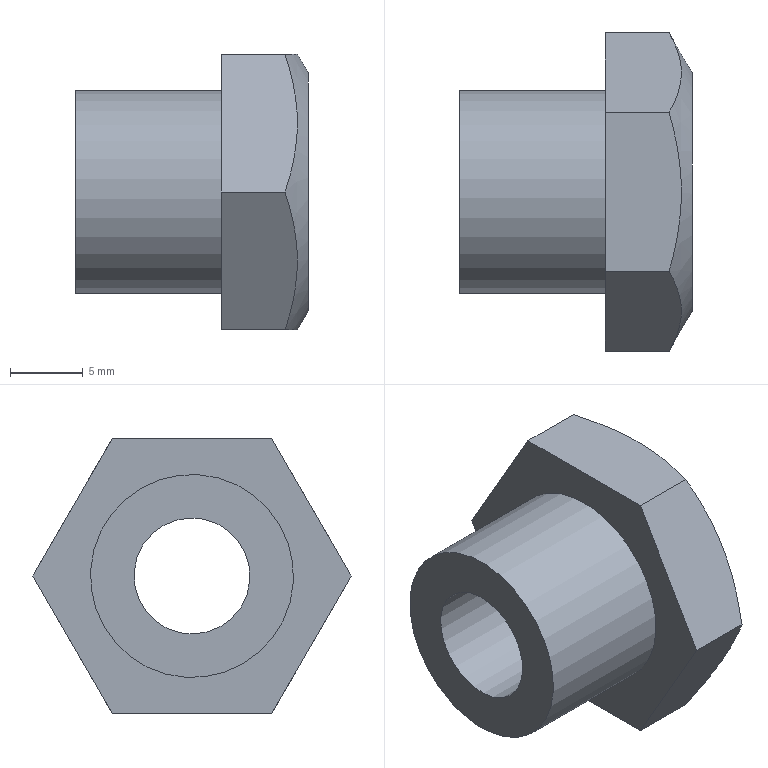Component | NX | OUTER_CASING_TUBE_CONNECTING_SCREW | 1 solid | 12 faces | box 16 x 21.94 x 19 mm | volume 2555 mm3 | plane 9 | cylinder 2 | cone 1 | commonest cylinder face diameters 14 x1 8 x1
STEP:
#1=CARTESIAN_POINT('',(0.,0.,0.));
#2=DIRECTION('',(0.,0.,1.));
#3=DIRECTION('',(1.,0.,0.));
#4=AXIS2_PLACEMENT_3D('',#1,#2,#3);
#5=CARTESIAN_POINT('',(-38.73,-48.,41.964));
#6=VERTEX_POINT('',#5);
#7=CARTESIAN_POINT('',(-38.73,-52.,35.036));
#8=VERTEX_POINT('',#7);
#9=CARTESIAN_POINT('',(-38.73,-50.,38.5));
#10=DIRECTION('',(1.,0.,0.));
#11=DIRECTION('',(0.,0.5,0.866));
#12=AXIS2_PLACEMENT_3D('',#9,#10,#11);
#13=CIRCLE('',#12,4.);
#14=CARTESIAN_POINT('',(-38.73,-50.,38.5));
#15=DIRECTION('',(-1.,0.,0.));
#16=DIRECTION('',(0.,0.5,0.866));
#17=AXIS2_PLACEMENT_3D('',#14,#15,#16);
#18=PLANE('',#17);
#19=CARTESIAN_POINT('',(4.,0.));
#20=CARTESIAN_POINT('',(4.,-6.928));
#21=CARTESIAN_POINT('',(-2.,-3.464));
#22=CARTESIAN_POINT('',(-8.,-0.));
#23=CARTESIAN_POINT('',(-2.,3.464));
#24=CARTESIAN_POINT('',(4.,6.928));
#25=CARTESIAN_POINT('',(4.,0.));
#26=(BOUNDED_CURVE()B_SPLINE_CURVE(2,(#19,#20,#21,#22,#23,#24,#25),.UNSPECIFIED.,.T.,.F.)B_SPLINE_CURVE_WITH_KNOTS((1,2,2,2,2,1),(-2.094,0.,2.094,4.189,6.283,8.378),.UNSPECIFIED.)CURVE()GEOMETRIC_REPRESENTATION_ITEM()RATIONAL_B_SPLINE_CURVE((1.,0.5,1.,0.5,1.,0.5,1.))REPRESENTATION_ITEM(''));
#27=(GEOMETRIC_REPRESENTATION_CONTEXT(2)PARAMETRIC_REPRESENTATION_CONTEXT()REPRESENTATION_CONTEXT('',''));
#28=DEFINITIONAL_REPRESENTATION('',(#26),#27);
#29=PCURVE('',#18,#28);
#30=CARTESIAN_POINT('',(-44.23,-50.,38.5));
#31=DIRECTION('',(1.,0.,0.));
#32=DIRECTION('',(0.,-0.5,-0.866));
#33=AXIS2_PLACEMENT_3D('',#30,#31,#32);
#34=CYLINDRICAL_SURFACE('',#33,4.);
#35=CARTESIAN_POINT('',(3.142,5.5));
#36=DIRECTION('',(1.,0.));
#37=VECTOR('',#36,1.);
#38=LINE('',#35,#37);
#39=(GEOMETRIC_REPRESENTATION_CONTEXT(2)PARAMETRIC_REPRESENTATION_CONTEXT()REPRESENTATION_CONTEXT('',''));
#40=DEFINITIONAL_REPRESENTATION('',(#38),#39);
#41=PCURVE('',#34,#40);
#42=SURFACE_CURVE('',#13,(#29,#41),.PCURVE_S1.);
#43=EDGE_CURVE('',#6,#8,#42,.T.);
#44=ORIENTED_EDGE('',*,*,#43,.T.);
#45=CARTESIAN_POINT('',(-38.73,-50.,38.5));
#46=DIRECTION('',(1.,0.,0.));
#47=DIRECTION('',(0.,0.5,0.866));
#48=AXIS2_PLACEMENT_3D('',#45,#46,#47);
#49=CIRCLE('',#48,4.);
#50=CARTESIAN_POINT('',(4.,0.));
#51=CARTESIAN_POINT('',(4.,-6.928));
#52=CARTESIAN_POINT('',(-2.,-3.464));
#53=CARTESIAN_POINT('',(-8.,-0.));
#54=CARTESIAN_POINT('',(-2.,3.464));
#55=CARTESIAN_POINT('',(4.,6.928));
#56=CARTESIAN_POINT('',(4.,0.));
#57=(BOUNDED_CURVE()B_SPLINE_CURVE(2,(#50,#51,#52,#53,#54,#55,#56),.UNSPECIFIED.,.T.,.F.)B_SPLINE_CURVE_WITH_KNOTS((1,2,2,2,2,1),(-2.094,0.,2.094,4.189,6.283,8.378),.UNSPECIFIED.)CURVE()GEOMETRIC_REPRESENTATION_ITEM()RATIONAL_B_SPLINE_CURVE((1.,0.5,1.,0.5,1.,0.5,1.))REPRESENTATION_ITEM(''));
#58=(GEOMETRIC_REPRESENTATION_CONTEXT(2)PARAMETRIC_REPRESENTATION_CONTEXT()REPRESENTATION_CONTEXT('',''));
#59=DEFINITIONAL_REPRESENTATION('',(#57),#58);
#60=PCURVE('',#18,#59);
#61=CARTESIAN_POINT('',(-3.142,5.5));
#62=DIRECTION('',(1.,0.));
#63=VECTOR('',#62,1.);
#64=LINE('',#61,#63);
#65=(GEOMETRIC_REPRESENTATION_CONTEXT(2)PARAMETRIC_REPRESENTATION_CONTEXT()REPRESENTATION_CONTEXT('',''));
#66=DEFINITIONAL_REPRESENTATION('',(#64),#65);
#67=PCURVE('',#34,#66);
#68=SURFACE_CURVE('',#49,(#60,#67),.PCURVE_S1.);
#69=EDGE_CURVE('',#8,#6,#68,.T.);
#70=ORIENTED_EDGE('',*,*,#69,.T.);
#71=EDGE_LOOP('',(#44,#70));
#72=FACE_BOUND('',#71,.T.);
#73=CARTESIAN_POINT('',(-38.73,-53.5,32.438));
#74=VERTEX_POINT('',#73);
#75=CARTESIAN_POINT('',(-38.73,-50.,38.5));
#76=DIRECTION('',(1.,0.,0.));
#77=DIRECTION('',(0.,-0.5,-0.866));
#78=AXIS2_PLACEMENT_3D('',#75,#76,#77);
#79=CIRCLE('',#78,7.);
#80=CARTESIAN_POINT('',(-7.,0.));
#81=CARTESIAN_POINT('',(-7.,12.124));
#82=CARTESIAN_POINT('',(3.5,6.062));
#83=CARTESIAN_POINT('',(14.,-0.));
#84=CARTESIAN_POINT('',(3.5,-6.062));
#85=CARTESIAN_POINT('',(-7.,-12.124));
#86=CARTESIAN_POINT('',(-7.,0.));
#87=(BOUNDED_CURVE()B_SPLINE_CURVE(2,(#80,#81,#82,#83,#84,#85,#86),.UNSPECIFIED.,.T.,.F.)B_SPLINE_CURVE_WITH_KNOTS((1,2,2,2,2,1),(-2.094,0.,2.094,4.189,6.283,8.378),.UNSPECIFIED.)CURVE()GEOMETRIC_REPRESENTATION_ITEM()RATIONAL_B_SPLINE_CURVE((1.,0.5,1.,0.5,1.,0.5,1.))REPRESENTATION_ITEM(''));
#88=(GEOMETRIC_REPRESENTATION_CONTEXT(2)PARAMETRIC_REPRESENTATION_CONTEXT()REPRESENTATION_CONTEXT('',''));
#89=DEFINITIONAL_REPRESENTATION('',(#87),#88);
#90=PCURVE('',#18,#89);
#91=CARTESIAN_POINT('',(-38.73,-50.,38.5));
#92=DIRECTION('',(1.,0.,0.));
#93=DIRECTION('',(0.,-0.5,-0.866));
#94=AXIS2_PLACEMENT_3D('',#91,#92,#93);
#95=CYLINDRICAL_SURFACE('',#94,7.);
#96=CARTESIAN_POINT('',(0.,0.));
#97=DIRECTION('',(1.,0.));
#98=VECTOR('',#97,1.);
#99=LINE('',#96,#98);
#100=(GEOMETRIC_REPRESENTATION_CONTEXT(2)PARAMETRIC_REPRESENTATION_CONTEXT()REPRESENTATION_CONTEXT('',''));
#101=DEFINITIONAL_REPRESENTATION('',(#99),#100);
#102=PCURVE('',#95,#101);
#103=SURFACE_CURVE('',#79,(#90,#102),.PCURVE_S1.);
#104=EDGE_CURVE('',#74,#74,#103,.T.);
#105=ORIENTED_EDGE('',*,*,#104,.F.);
#106=EDGE_LOOP('',(#105));
#107=FACE_BOUND('',#106,.T.);
#108=ADVANCED_FACE('',(#72,#107),#18,.T.);
#109=CARTESIAN_POINT('',(-28.73,-53.5,32.438));
#110=VERTEX_POINT('',#109);
#111=CARTESIAN_POINT('',(-28.73,-50.,38.5));
#112=DIRECTION('',(-1.,0.,0.));
#113=DIRECTION('',(0.,-0.5,-0.866));
#114=AXIS2_PLACEMENT_3D('',#111,#112,#113);
#115=CIRCLE('',#114,7.);
#116=CARTESIAN_POINT('',(6.283,10.));
#117=DIRECTION('',(-1.,0.));
#118=VECTOR('',#117,1.);
#119=LINE('',#116,#118);
#120=(GEOMETRIC_REPRESENTATION_CONTEXT(2)PARAMETRIC_REPRESENTATION_CONTEXT()REPRESENTATION_CONTEXT('',''));
#121=DEFINITIONAL_REPRESENTATION('',(#119),#120);
#122=PCURVE('',#95,#121);
#123=CARTESIAN_POINT('',(-28.73,-50.,38.5));
#124=DIRECTION('',(-1.,0.,0.));
#125=DIRECTION('',(0.,0.5,0.866));
#126=AXIS2_PLACEMENT_3D('',#123,#124,#125);
#127=PLANE('',#126);
#128=CARTESIAN_POINT('',(0.,0.));
#129=DIRECTION('',(-1.,0.));
#130=AXIS2_PLACEMENT_2D('',#128,#129);
#131=CIRCLE('',#130,7.);
#132=(GEOMETRIC_REPRESENTATION_CONTEXT(2)PARAMETRIC_REPRESENTATION_CONTEXT()REPRESENTATION_CONTEXT('',''));
#133=DEFINITIONAL_REPRESENTATION('',(#131),#132);
#134=PCURVE('',#127,#133);
#135=SURFACE_CURVE('',#115,(#122,#134),.PCURVE_S1.);
#136=EDGE_CURVE('',#110,#110,#135,.T.);
#137=ORIENTED_EDGE('',*,*,#136,.T.);
#138=CARTESIAN_POINT('',(-38.73,-53.5,32.438));
#139=CARTESIAN_POINT('',(-28.73,-53.5,32.438));
#140=B_SPLINE_CURVE_WITH_KNOTS('',1,(#138,#139),.UNSPECIFIED.,.F.,.F.,(2,2),(0.,10.),.PIECEWISE_BEZIER_KNOTS.);
#141=CARTESIAN_POINT('',(0.,0.));
#142=DIRECTION('',(0.,1.));
#143=VECTOR('',#142,1.);
#144=LINE('',#141,#143);
#145=(GEOMETRIC_REPRESENTATION_CONTEXT(2)PARAMETRIC_REPRESENTATION_CONTEXT()REPRESENTATION_CONTEXT('',''));
#146=DEFINITIONAL_REPRESENTATION('',(#144),#145);
#147=PCURVE('',#95,#146);
#148=CARTESIAN_POINT('',(6.283,0.));
#149=DIRECTION('',(0.,1.));
#150=VECTOR('',#149,1.);
#151=LINE('',#148,#150);
#152=(GEOMETRIC_REPRESENTATION_CONTEXT(2)PARAMETRIC_REPRESENTATION_CONTEXT()REPRESENTATION_CONTEXT('',''));
#153=DEFINITIONAL_REPRESENTATION('',(#151),#152);
#154=PCURVE('',#95,#153);
#155=SEAM_CURVE('',#140,(#147,#154),.PCURVE_S1.);
#156=EDGE_CURVE('',#74,#110,#155,.T.);
#157=ORIENTED_EDGE('',*,*,#156,.F.);
#158=ORIENTED_EDGE('',*,*,#104,.T.);
#159=ORIENTED_EDGE('',*,*,#156,.T.);
#160=EDGE_LOOP('',(#137,#157,#158,#159));
#161=FACE_BOUND('',#160,.T.);
#162=ADVANCED_FACE('',(#161),#95,.T.);
#163=CARTESIAN_POINT('',(-24.314,-55.485,29.));
#164=VERTEX_POINT('',#163);
#165=CARTESIAN_POINT('',(-24.314,-44.515,29.));
#166=VERTEX_POINT('',#165);
#167=CARTESIAN_POINT('',(-24.314,-55.485,29.));
#168=CARTESIAN_POINT('',(-23.797,-53.694,29.));
#169=CARTESIAN_POINT('',(-23.466,-51.876,29.));
#170=CARTESIAN_POINT('',(-23.464,-48.145,29.));
#171=CARTESIAN_POINT('',(-23.796,-46.309,29.));
#172=CARTESIAN_POINT('',(-24.314,-44.515,29.));
#173=B_SPLINE_CURVE_WITH_KNOTS('',3,(#167,#168,#169,#170,#171,#172),.UNSPECIFIED.,.F.,.F.,(4,2,4),(0.,0.5,1.),.UNSPECIFIED.);
#174=CARTESIAN_POINT('',(-22.73,-44.515,29.));
#175=DIRECTION('',(0.,0.,-1.));
#176=DIRECTION('',(0.,1.,0.));
#177=AXIS2_PLACEMENT_3D('',#174,#175,#176);
#178=PLANE('',#177);
#179=CARTESIAN_POINT('',(-10.97,-1.583));
#180=CARTESIAN_POINT('',(-9.179,-1.066));
#181=CARTESIAN_POINT('',(-7.361,-0.736));
#182=CARTESIAN_POINT('',(-3.63,-0.7336));
#183=CARTESIAN_POINT('',(-1.793,-1.066));
#184=CARTESIAN_POINT('',(0.,-1.583));
#185=B_SPLINE_CURVE_WITH_KNOTS('',3,(#179,#180,#181,#182,#183,#184),.UNSPECIFIED.,.F.,.F.,(4,2,4),(0.,0.5,1.),.UNSPECIFIED.);
#186=(GEOMETRIC_REPRESENTATION_CONTEXT(2)PARAMETRIC_REPRESENTATION_CONTEXT()REPRESENTATION_CONTEXT('',''));
#187=DEFINITIONAL_REPRESENTATION('',(#185),#186);
#188=PCURVE('',#178,#187);
#189=CARTESIAN_POINT('',(-22.73,-50.,38.5));
#190=DIRECTION('',(-1.,0.,0.));
#191=DIRECTION('',(0.,0.5,0.866));
#192=AXIS2_PLACEMENT_3D('',#189,#190,#191);
#193=CONICAL_SURFACE('',#192,8.227,1.047);
#194=CARTESIAN_POINT('',(3.142,1.583));
#195=CARTESIAN_POINT('',(3.129,1.536));
#196=CARTESIAN_POINT('',(3.102,1.445));
#197=CARTESIAN_POINT('',(3.061,1.319));
#198=CARTESIAN_POINT('',(3.018,1.202));
#199=CARTESIAN_POINT('',(2.973,1.097));
#200=CARTESIAN_POINT('',(2.926,1.004));
#201=CARTESIAN_POINT('',(2.878,0.9237));
#202=CARTESIAN_POINT('',(2.828,0.8564));
#203=CARTESIAN_POINT('',(2.777,0.8031));
#204=CARTESIAN_POINT('',(2.725,0.7642));
#205=CARTESIAN_POINT('',(2.673,0.7404));
#206=CARTESIAN_POINT('',(2.619,0.7322));
#207=CARTESIAN_POINT('',(2.566,0.7398));
#208=CARTESIAN_POINT('',(2.513,0.7631));
#209=CARTESIAN_POINT('',(2.46,0.8015));
#210=CARTESIAN_POINT('',(2.409,0.8547));
#211=CARTESIAN_POINT('',(2.359,0.9219));
#212=CARTESIAN_POINT('',(2.311,1.003));
#213=CARTESIAN_POINT('',(2.264,1.096));
#214=CARTESIAN_POINT('',(2.218,1.201));
#215=CARTESIAN_POINT('',(2.175,1.318));
#216=CARTESIAN_POINT('',(2.134,1.445));
#217=CARTESIAN_POINT('',(2.107,1.536));
#218=CARTESIAN_POINT('',(2.094,1.583));
#219=B_SPLINE_CURVE_WITH_KNOTS('',3,(#194,#195,#196,#197,#198,#199,#200,#201,#202,#203,#204,#205,#206,#207,#208,#209,#210,#211,#212,#213,#214,#215,#216,#217,#218),.UNSPECIFIED.,.F.,.F.,(4,1,1,1,1,1,1,1,1,1,1,1,1,1,1,1,1,1,1,1,1,1,4),(0.,0.04545,0.09091,0.1364,0.1818,0.2273,0.2727,0.3182,0.3636,0.4091,0.4545,0.5,0.5455,0.5909,0.6364,0.6818,0.7273,0.7727,0.8182,0.8636,0.9091,0.9545,1.),.QUASI_UNIFORM_KNOTS.);
#220=(GEOMETRIC_REPRESENTATION_CONTEXT(2)PARAMETRIC_REPRESENTATION_CONTEXT()REPRESENTATION_CONTEXT('',''));
#221=DEFINITIONAL_REPRESENTATION('',(#219),#220);
#222=PCURVE('',#193,#221);
#223=SURFACE_CURVE('',#173,(#188,#222),.PCURVE_S1.);
#224=EDGE_CURVE('',#164,#166,#223,.T.);
#225=ORIENTED_EDGE('',*,*,#224,.F.);
#226=CARTESIAN_POINT('',(-28.73,-55.485,29.));
#227=VERTEX_POINT('',#226);
#228=CARTESIAN_POINT('',(-22.73,-55.485,29.));
#229=DIRECTION('',(-1.,0.,0.));
#230=VECTOR('',#229,1.);
#231=LINE('',#228,#230);
#232=CARTESIAN_POINT('',(-10.97,0.));
#233=DIRECTION('',(0.,-1.));
#234=VECTOR('',#233,1.);
#235=LINE('',#232,#234);
#236=(GEOMETRIC_REPRESENTATION_CONTEXT(2)PARAMETRIC_REPRESENTATION_CONTEXT()REPRESENTATION_CONTEXT('',''));
#237=DEFINITIONAL_REPRESENTATION('',(#235),#236);
#238=PCURVE('',#178,#237);
#239=CARTESIAN_POINT('',(-22.73,-55.485,29.));
#240=DIRECTION('',(0.,-0.866,-0.5));
#241=DIRECTION('',(0.,0.5,-0.866));
#242=AXIS2_PLACEMENT_3D('',#239,#240,#241);
#243=PLANE('',#242);
#244=CARTESIAN_POINT('',(0.,0.));
#245=DIRECTION('',(0.,-1.));
#246=VECTOR('',#245,1.);
#247=LINE('',#244,#246);
#248=(GEOMETRIC_REPRESENTATION_CONTEXT(2)PARAMETRIC_REPRESENTATION_CONTEXT()REPRESENTATION_CONTEXT('',''));
#249=DEFINITIONAL_REPRESENTATION('',(#247),#248);
#250=PCURVE('',#243,#249);
#251=SURFACE_CURVE('',#231,(#238,#250),.PCURVE_S1.);
#252=EDGE_CURVE('',#164,#227,#251,.T.);
#253=ORIENTED_EDGE('',*,*,#252,.T.);
#254=CARTESIAN_POINT('',(-28.73,-44.515,29.));
#255=VERTEX_POINT('',#254);
#256=CARTESIAN_POINT('',(-28.73,-44.515,29.));
#257=DIRECTION('',(0.,-1.,-0.));
#258=VECTOR('',#257,1.);
#259=LINE('',#256,#258);
#260=CARTESIAN_POINT('',(0.,-6.));
#261=DIRECTION('',(-1.,0.));
#262=VECTOR('',#261,1.);
#263=LINE('',#260,#262);
#264=(GEOMETRIC_REPRESENTATION_CONTEXT(2)PARAMETRIC_REPRESENTATION_CONTEXT()REPRESENTATION_CONTEXT('',''));
#265=DEFINITIONAL_REPRESENTATION('',(#263),#264);
#266=PCURVE('',#178,#265);
#267=CARTESIAN_POINT('',(-5.485,9.5));
#268=DIRECTION('',(-0.5,-0.866));
#269=VECTOR('',#268,1.);
#270=LINE('',#267,#269);
#271=(GEOMETRIC_REPRESENTATION_CONTEXT(2)PARAMETRIC_REPRESENTATION_CONTEXT()REPRESENTATION_CONTEXT('',''));
#272=DEFINITIONAL_REPRESENTATION('',(#270),#271);
#273=PCURVE('',#127,#272);
#274=SURFACE_CURVE('',#259,(#266,#273),.PCURVE_S1.);
#275=EDGE_CURVE('',#255,#227,#274,.T.);
#276=ORIENTED_EDGE('',*,*,#275,.F.);
#277=CARTESIAN_POINT('',(-22.73,-44.515,29.));
#278=DIRECTION('',(-1.,0.,0.));
#279=VECTOR('',#278,1.);
#280=LINE('',#277,#279);
#281=CARTESIAN_POINT('',(0.,0.));
#282=DIRECTION('',(0.,-1.));
#283=VECTOR('',#282,1.);
#284=LINE('',#281,#283);
#285=(GEOMETRIC_REPRESENTATION_CONTEXT(2)PARAMETRIC_REPRESENTATION_CONTEXT()REPRESENTATION_CONTEXT('',''));
#286=DEFINITIONAL_REPRESENTATION('',(#284),#285);
#287=PCURVE('',#178,#286);
#288=CARTESIAN_POINT('',(-22.73,-39.03,38.5));
#289=DIRECTION('',(0.,0.866,-0.5));
#290=DIRECTION('',(0.,0.5,0.866));
#291=AXIS2_PLACEMENT_3D('',#288,#289,#290);
#292=PLANE('',#291);
#293=CARTESIAN_POINT('',(-10.97,0.));
#294=DIRECTION('',(0.,-1.));
#295=VECTOR('',#294,1.);
#296=LINE('',#293,#295);
#297=(GEOMETRIC_REPRESENTATION_CONTEXT(2)PARAMETRIC_REPRESENTATION_CONTEXT()REPRESENTATION_CONTEXT('',''));
#298=DEFINITIONAL_REPRESENTATION('',(#296),#297);
#299=PCURVE('',#292,#298);
#300=SURFACE_CURVE('',#280,(#287,#299),.PCURVE_S1.);
#301=EDGE_CURVE('',#166,#255,#300,.T.);
#302=ORIENTED_EDGE('',*,*,#301,.F.);
#303=EDGE_LOOP('',(#225,#253,#276,#302));
#304=FACE_BOUND('',#303,.T.);
#305=ADVANCED_FACE('',(#304),#178,.T.);
#306=CARTESIAN_POINT('',(-24.314,-60.97,38.5));
#307=VERTEX_POINT('',#306);
#308=CARTESIAN_POINT('',(-24.314,-60.97,38.5));
#309=CARTESIAN_POINT('',(-23.797,-60.074,36.949));
#310=CARTESIAN_POINT('',(-23.466,-59.165,35.374));
#311=CARTESIAN_POINT('',(-23.464,-57.3,32.144));
#312=CARTESIAN_POINT('',(-23.796,-56.382,30.553));
#313=CARTESIAN_POINT('',(-24.314,-55.485,29.));
#314=B_SPLINE_CURVE_WITH_KNOTS('',3,(#308,#309,#310,#311,#312,#313),.UNSPECIFIED.,.F.,.F.,(4,2,4),(0.,0.5,1.),.UNSPECIFIED.);
#315=CARTESIAN_POINT('',(-10.97,-1.583));
#316=CARTESIAN_POINT('',(-9.179,-1.066));
#317=CARTESIAN_POINT('',(-7.361,-0.736));
#318=CARTESIAN_POINT('',(-3.63,-0.7336));
#319=CARTESIAN_POINT('',(-1.793,-1.066));
#320=CARTESIAN_POINT('',(0.,-1.583));
#321=B_SPLINE_CURVE_WITH_KNOTS('',3,(#315,#316,#317,#318,#319,#320),.UNSPECIFIED.,.F.,.F.,(4,2,4),(0.,0.5,1.),.UNSPECIFIED.);
#322=(GEOMETRIC_REPRESENTATION_CONTEXT(2)PARAMETRIC_REPRESENTATION_CONTEXT()REPRESENTATION_CONTEXT('',''));
#323=DEFINITIONAL_REPRESENTATION('',(#321),#322);
#324=PCURVE('',#243,#323);
#325=CARTESIAN_POINT('',(4.189,1.583));
#326=CARTESIAN_POINT('',(4.176,1.536));
#327=CARTESIAN_POINT('',(4.15,1.445));
#328=CARTESIAN_POINT('',(4.108,1.319));
#329=CARTESIAN_POINT('',(4.065,1.202));
#330=CARTESIAN_POINT('',(4.02,1.097));
#331=CARTESIAN_POINT('',(3.974,1.004));
#332=CARTESIAN_POINT('',(3.925,0.9237));
#333=CARTESIAN_POINT('',(3.876,0.8564));
#334=CARTESIAN_POINT('',(3.825,0.8031));
#335=CARTESIAN_POINT('',(3.773,0.7642));
#336=CARTESIAN_POINT('',(3.72,0.7404));
#337=CARTESIAN_POINT('',(3.666,0.7322));
#338=CARTESIAN_POINT('',(3.613,0.7398));
#339=CARTESIAN_POINT('',(3.56,0.7631));
#340=CARTESIAN_POINT('',(3.507,0.8015));
#341=CARTESIAN_POINT('',(3.456,0.8547));
#342=CARTESIAN_POINT('',(3.406,0.9219));
#343=CARTESIAN_POINT('',(3.358,1.003));
#344=CARTESIAN_POINT('',(3.311,1.096));
#345=CARTESIAN_POINT('',(3.266,1.201));
#346=CARTESIAN_POINT('',(3.222,1.318));
#347=CARTESIAN_POINT('',(3.181,1.445));
#348=CARTESIAN_POINT('',(3.154,1.536));
#349=CARTESIAN_POINT('',(3.142,1.583));
#350=B_SPLINE_CURVE_WITH_KNOTS('',3,(#325,#326,#327,#328,#329,#330,#331,#332,#333,#334,#335,#336,#337,#338,#339,#340,#341,#342,#343,#344,#345,#346,#347,#348,#349),.UNSPECIFIED.,.F.,.F.,(4,1,1,1,1,1,1,1,1,1,1,1,1,1,1,1,1,1,1,1,1,1,4),(0.,0.04545,0.09091,0.1364,0.1818,0.2273,0.2727,0.3182,0.3636,0.4091,0.4545,0.5,0.5455,0.5909,0.6364,0.6818,0.7273,0.7727,0.8182,0.8636,0.9091,0.9545,1.),.QUASI_UNIFORM_KNOTS.);
#351=(GEOMETRIC_REPRESENTATION_CONTEXT(2)PARAMETRIC_REPRESENTATION_CONTEXT()REPRESENTATION_CONTEXT('',''));
#352=DEFINITIONAL_REPRESENTATION('',(#350),#351);
#353=PCURVE('',#193,#352);
#354=SURFACE_CURVE('',#314,(#324,#353),.PCURVE_S1.);
#355=EDGE_CURVE('',#307,#164,#354,.T.);
#356=ORIENTED_EDGE('',*,*,#355,.F.);
#357=CARTESIAN_POINT('',(-28.73,-60.97,38.5));
#358=VERTEX_POINT('',#357);
#359=CARTESIAN_POINT('',(-22.73,-60.97,38.5));
#360=DIRECTION('',(-1.,0.,0.));
#361=VECTOR('',#360,1.);
#362=LINE('',#359,#361);
#363=CARTESIAN_POINT('',(-10.97,0.));
#364=DIRECTION('',(0.,-1.));
#365=VECTOR('',#364,1.);
#366=LINE('',#363,#365);
#367=(GEOMETRIC_REPRESENTATION_CONTEXT(2)PARAMETRIC_REPRESENTATION_CONTEXT()REPRESENTATION_CONTEXT('',''));
#368=DEFINITIONAL_REPRESENTATION('',(#366),#367);
#369=PCURVE('',#243,#368);
#370=CARTESIAN_POINT('',(-22.73,-60.97,38.5));
#371=DIRECTION('',(0.,-0.866,0.5));
#372=DIRECTION('',(0.,-0.5,-0.866));
#373=AXIS2_PLACEMENT_3D('',#370,#371,#372);
#374=PLANE('',#373);
#375=CARTESIAN_POINT('',(0.,0.));
#376=DIRECTION('',(0.,-1.));
#377=VECTOR('',#376,1.);
#378=LINE('',#375,#377);
#379=(GEOMETRIC_REPRESENTATION_CONTEXT(2)PARAMETRIC_REPRESENTATION_CONTEXT()REPRESENTATION_CONTEXT('',''));
#380=DEFINITIONAL_REPRESENTATION('',(#378),#379);
#381=PCURVE('',#374,#380);
#382=SURFACE_CURVE('',#362,(#369,#381),.PCURVE_S1.);
#383=EDGE_CURVE('',#307,#358,#382,.T.);
#384=ORIENTED_EDGE('',*,*,#383,.T.);
#385=CARTESIAN_POINT('',(-28.73,-55.485,29.));
#386=DIRECTION('',(0.,-0.5,0.866));
#387=VECTOR('',#386,1.);
#388=LINE('',#385,#387);
#389=CARTESIAN_POINT('',(0.,-6.));
#390=DIRECTION('',(-1.,0.));
#391=VECTOR('',#390,1.);
#392=LINE('',#389,#391);
#393=(GEOMETRIC_REPRESENTATION_CONTEXT(2)PARAMETRIC_REPRESENTATION_CONTEXT()REPRESENTATION_CONTEXT('',''));
#394=DEFINITIONAL_REPRESENTATION('',(#392),#393);
#395=PCURVE('',#243,#394);
#396=CARTESIAN_POINT('',(-10.97,0.));
#397=DIRECTION('',(0.5,-0.866));
#398=VECTOR('',#397,1.);
#399=LINE('',#396,#398);
#400=(GEOMETRIC_REPRESENTATION_CONTEXT(2)PARAMETRIC_REPRESENTATION_CONTEXT()REPRESENTATION_CONTEXT('',''));
#401=DEFINITIONAL_REPRESENTATION('',(#399),#400);
#402=PCURVE('',#127,#401);
#403=SURFACE_CURVE('',#388,(#395,#402),.PCURVE_S1.);
#404=EDGE_CURVE('',#227,#358,#403,.T.);
#405=ORIENTED_EDGE('',*,*,#404,.F.);
#406=ORIENTED_EDGE('',*,*,#252,.F.);
#407=EDGE_LOOP('',(#356,#384,#405,#406));
#408=FACE_BOUND('',#407,.T.);
#409=ADVANCED_FACE('',(#408),#243,.T.);
#410=CARTESIAN_POINT('',(-24.314,-55.485,48.));
#411=VERTEX_POINT('',#410);
#412=CARTESIAN_POINT('',(-24.314,-55.485,48.));
#413=CARTESIAN_POINT('',(-23.799,-56.377,46.455));
#414=CARTESIAN_POINT('',(-23.465,-57.301,44.854));
#415=CARTESIAN_POINT('',(-23.465,-59.155,41.643));
#416=CARTESIAN_POINT('',(-23.802,-60.083,40.036));
#417=CARTESIAN_POINT('',(-24.314,-60.97,38.5));
#418=B_SPLINE_CURVE_WITH_KNOTS('',3,(#412,#413,#414,#415,#416,#417),.UNSPECIFIED.,.F.,.F.,(4,2,4),(0.,0.5,1.),.UNSPECIFIED.);
#419=CARTESIAN_POINT('',(-10.97,-1.583));
#420=CARTESIAN_POINT('',(-9.186,-1.068));
#421=CARTESIAN_POINT('',(-7.337,-0.7347));
#422=CARTESIAN_POINT('',(-3.63,-0.735));
#423=CARTESIAN_POINT('',(-1.773,-1.071));
#424=CARTESIAN_POINT('',(0.,-1.583));
#425=B_SPLINE_CURVE_WITH_KNOTS('',3,(#419,#420,#421,#422,#423,#424),.UNSPECIFIED.,.F.,.F.,(4,2,4),(0.,0.5,1.),.UNSPECIFIED.);
#426=(GEOMETRIC_REPRESENTATION_CONTEXT(2)PARAMETRIC_REPRESENTATION_CONTEXT()REPRESENTATION_CONTEXT('',''));
#427=DEFINITIONAL_REPRESENTATION('',(#425),#426);
#428=PCURVE('',#374,#427);
#429=CARTESIAN_POINT('',(5.236,1.583));
#430=CARTESIAN_POINT('',(5.223,1.537));
#431=CARTESIAN_POINT('',(5.197,1.446));
#432=CARTESIAN_POINT('',(5.156,1.319));
#433=CARTESIAN_POINT('',(5.112,1.202));
#434=CARTESIAN_POINT('',(5.067,1.097));
#435=CARTESIAN_POINT('',(5.02,1.003));
#436=CARTESIAN_POINT('',(4.972,0.9227));
#437=CARTESIAN_POINT('',(4.922,0.8553));
#438=CARTESIAN_POINT('',(4.87,0.802));
#439=CARTESIAN_POINT('',(4.818,0.7634));
#440=CARTESIAN_POINT('',(4.765,0.74));
#441=CARTESIAN_POINT('',(4.712,0.7322));
#442=CARTESIAN_POINT('',(4.659,0.7402));
#443=CARTESIAN_POINT('',(4.606,0.7637));
#444=CARTESIAN_POINT('',(4.554,0.8025));
#445=CARTESIAN_POINT('',(4.503,0.856));
#446=CARTESIAN_POINT('',(4.453,0.9236));
#447=CARTESIAN_POINT('',(4.404,1.005));
#448=CARTESIAN_POINT('',(4.357,1.098));
#449=CARTESIAN_POINT('',(4.312,1.204));
#450=CARTESIAN_POINT('',(4.269,1.32));
#451=CARTESIAN_POINT('',(4.228,1.446));
#452=CARTESIAN_POINT('',(4.202,1.537));
#453=CARTESIAN_POINT('',(4.189,1.583));
#454=B_SPLINE_CURVE_WITH_KNOTS('',3,(#429,#430,#431,#432,#433,#434,#435,#436,#437,#438,#439,#440,#441,#442,#443,#444,#445,#446,#447,#448,#449,#450,#451,#452,#453),.UNSPECIFIED.,.F.,.F.,(4,1,1,1,1,1,1,1,1,1,1,1,1,1,1,1,1,1,1,1,1,1,4),(0.,0.04545,0.09091,0.1364,0.1818,0.2273,0.2727,0.3182,0.3636,0.4091,0.4545,0.5,0.5455,0.5909,0.6364,0.6818,0.7273,0.7727,0.8182,0.8636,0.9091,0.9545,1.),.QUASI_UNIFORM_KNOTS.);
#455=(GEOMETRIC_REPRESENTATION_CONTEXT(2)PARAMETRIC_REPRESENTATION_CONTEXT()REPRESENTATION_CONTEXT('',''));
#456=DEFINITIONAL_REPRESENTATION('',(#454),#455);
#457=PCURVE('',#193,#456);
#458=SURFACE_CURVE('',#418,(#428,#457),.PCURVE_S1.);
#459=EDGE_CURVE('',#411,#307,#458,.T.);
#460=ORIENTED_EDGE('',*,*,#459,.F.);
#461=CARTESIAN_POINT('',(-28.73,-55.485,48.));
#462=VERTEX_POINT('',#461);
#463=CARTESIAN_POINT('',(-22.73,-55.485,48.));
#464=DIRECTION('',(-1.,0.,0.));
#465=VECTOR('',#464,1.);
#466=LINE('',#463,#465);
#467=CARTESIAN_POINT('',(-10.97,0.));
#468=DIRECTION('',(0.,-1.));
#469=VECTOR('',#468,1.);
#470=LINE('',#467,#469);
#471=(GEOMETRIC_REPRESENTATION_CONTEXT(2)PARAMETRIC_REPRESENTATION_CONTEXT()REPRESENTATION_CONTEXT('',''));
#472=DEFINITIONAL_REPRESENTATION('',(#470),#471);
#473=PCURVE('',#374,#472);
#474=CARTESIAN_POINT('',(-22.73,-55.485,48.));
#475=DIRECTION('',(0.,-0.,1.));
#476=DIRECTION('',(0.,-1.,-0.));
#477=AXIS2_PLACEMENT_3D('',#474,#475,#476);
#478=PLANE('',#477);
#479=CARTESIAN_POINT('',(0.,0.));
#480=DIRECTION('',(0.,-1.));
#481=VECTOR('',#480,1.);
#482=LINE('',#479,#481);
#483=(GEOMETRIC_REPRESENTATION_CONTEXT(2)PARAMETRIC_REPRESENTATION_CONTEXT()REPRESENTATION_CONTEXT('',''));
#484=DEFINITIONAL_REPRESENTATION('',(#482),#483);
#485=PCURVE('',#478,#484);
#486=SURFACE_CURVE('',#466,(#473,#485),.PCURVE_S1.);
#487=EDGE_CURVE('',#411,#462,#486,.T.);
#488=ORIENTED_EDGE('',*,*,#487,.T.);
#489=CARTESIAN_POINT('',(-28.73,-60.97,38.5));
#490=DIRECTION('',(0.,0.5,0.866));
#491=VECTOR('',#490,1.);
#492=LINE('',#489,#491);
#493=CARTESIAN_POINT('',(0.,-6.));
#494=DIRECTION('',(-1.,0.));
#495=VECTOR('',#494,1.);
#496=LINE('',#493,#495);
#497=(GEOMETRIC_REPRESENTATION_CONTEXT(2)PARAMETRIC_REPRESENTATION_CONTEXT()REPRESENTATION_CONTEXT('',''));
#498=DEFINITIONAL_REPRESENTATION('',(#496),#497);
#499=PCURVE('',#374,#498);
#500=CARTESIAN_POINT('',(-5.485,-9.5));
#501=DIRECTION('',(1.,0.));
#502=VECTOR('',#501,1.);
#503=LINE('',#500,#502);
#504=(GEOMETRIC_REPRESENTATION_CONTEXT(2)PARAMETRIC_REPRESENTATION_CONTEXT()REPRESENTATION_CONTEXT('',''));
#505=DEFINITIONAL_REPRESENTATION('',(#503),#504);
#506=PCURVE('',#127,#505);
#507=SURFACE_CURVE('',#492,(#499,#506),.PCURVE_S1.);
#508=EDGE_CURVE('',#358,#462,#507,.T.);
#509=ORIENTED_EDGE('',*,*,#508,.F.);
#510=ORIENTED_EDGE('',*,*,#383,.F.);
#511=EDGE_LOOP('',(#460,#488,#509,#510));
#512=FACE_BOUND('',#511,.T.);
#513=ADVANCED_FACE('',(#512),#374,.T.);
#514=CARTESIAN_POINT('',(-24.314,-44.515,48.));
#515=VERTEX_POINT('',#514);
#516=CARTESIAN_POINT('',(-24.314,-44.515,48.));
#517=CARTESIAN_POINT('',(-23.797,-46.306,48.));
#518=CARTESIAN_POINT('',(-23.466,-48.124,48.));
#519=CARTESIAN_POINT('',(-23.464,-51.855,48.));
#520=CARTESIAN_POINT('',(-23.796,-53.691,48.));
#521=CARTESIAN_POINT('',(-24.314,-55.485,48.));
#522=B_SPLINE_CURVE_WITH_KNOTS('',3,(#516,#517,#518,#519,#520,#521),.UNSPECIFIED.,.F.,.F.,(4,2,4),(0.,0.5,1.),.UNSPECIFIED.);
#523=CARTESIAN_POINT('',(-10.97,-1.583));
#524=CARTESIAN_POINT('',(-9.179,-1.066));
#525=CARTESIAN_POINT('',(-7.361,-0.736));
#526=CARTESIAN_POINT('',(-3.63,-0.7336));
#527=CARTESIAN_POINT('',(-1.793,-1.066));
#528=CARTESIAN_POINT('',(0.,-1.583));
#529=B_SPLINE_CURVE_WITH_KNOTS('',3,(#523,#524,#525,#526,#527,#528),.UNSPECIFIED.,.F.,.F.,(4,2,4),(0.,0.5,1.),.UNSPECIFIED.);
#530=(GEOMETRIC_REPRESENTATION_CONTEXT(2)PARAMETRIC_REPRESENTATION_CONTEXT()REPRESENTATION_CONTEXT('',''));
#531=DEFINITIONAL_REPRESENTATION('',(#529),#530);
#532=PCURVE('',#478,#531);
#533=CARTESIAN_POINT('',(6.283,1.583));
#534=CARTESIAN_POINT('',(6.27,1.536));
#535=CARTESIAN_POINT('',(6.244,1.445));
#536=CARTESIAN_POINT('',(6.203,1.319));
#537=CARTESIAN_POINT('',(6.16,1.202));
#538=CARTESIAN_POINT('',(6.115,1.097));
#539=CARTESIAN_POINT('',(6.068,1.004));
#540=CARTESIAN_POINT('',(6.02,0.9237));
#541=CARTESIAN_POINT('',(5.97,0.8564));
#542=CARTESIAN_POINT('',(5.919,0.8031));
#543=CARTESIAN_POINT('',(5.867,0.7642));
#544=CARTESIAN_POINT('',(5.814,0.7404));
#545=CARTESIAN_POINT('',(5.761,0.7322));
#546=CARTESIAN_POINT('',(5.707,0.7398));
#547=CARTESIAN_POINT('',(5.654,0.7631));
#548=CARTESIAN_POINT('',(5.602,0.8015));
#549=CARTESIAN_POINT('',(5.551,0.8547));
#550=CARTESIAN_POINT('',(5.501,0.9219));
#551=CARTESIAN_POINT('',(5.452,1.003));
#552=CARTESIAN_POINT('',(5.405,1.096));
#553=CARTESIAN_POINT('',(5.36,1.201));
#554=CARTESIAN_POINT('',(5.317,1.318));
#555=CARTESIAN_POINT('',(5.275,1.445));
#556=CARTESIAN_POINT('',(5.249,1.536));
#557=CARTESIAN_POINT('',(5.236,1.583));
#558=B_SPLINE_CURVE_WITH_KNOTS('',3,(#533,#534,#535,#536,#537,#538,#539,#540,#541,#542,#543,#544,#545,#546,#547,#548,#549,#550,#551,#552,#553,#554,#555,#556,#557),.UNSPECIFIED.,.F.,.F.,(4,1,1,1,1,1,1,1,1,1,1,1,1,1,1,1,1,1,1,1,1,1,4),(0.,0.04545,0.09091,0.1364,0.1818,0.2273,0.2727,0.3182,0.3636,0.4091,0.4545,0.5,0.5455,0.5909,0.6364,0.6818,0.7273,0.7727,0.8182,0.8636,0.9091,0.9545,1.),.QUASI_UNIFORM_KNOTS.);
#559=(GEOMETRIC_REPRESENTATION_CONTEXT(2)PARAMETRIC_REPRESENTATION_CONTEXT()REPRESENTATION_CONTEXT('',''));
#560=DEFINITIONAL_REPRESENTATION('',(#558),#559);
#561=PCURVE('',#193,#560);
#562=SURFACE_CURVE('',#522,(#532,#561),.PCURVE_S1.);
#563=EDGE_CURVE('',#515,#411,#562,.T.);
#564=ORIENTED_EDGE('',*,*,#563,.F.);
#565=CARTESIAN_POINT('',(-28.73,-44.515,48.));
#566=VERTEX_POINT('',#565);
#567=CARTESIAN_POINT('',(-22.73,-44.515,48.));
#568=DIRECTION('',(-1.,0.,0.));
#569=VECTOR('',#568,1.);
#570=LINE('',#567,#569);
#571=CARTESIAN_POINT('',(-10.97,0.));
#572=DIRECTION('',(0.,-1.));
#573=VECTOR('',#572,1.);
#574=LINE('',#571,#573);
#575=(GEOMETRIC_REPRESENTATION_CONTEXT(2)PARAMETRIC_REPRESENTATION_CONTEXT()REPRESENTATION_CONTEXT('',''));
#576=DEFINITIONAL_REPRESENTATION('',(#574),#575);
#577=PCURVE('',#478,#576);
#578=CARTESIAN_POINT('',(-22.73,-44.515,48.));
#579=DIRECTION('',(0.,0.866,0.5));
#580=DIRECTION('',(0.,-0.5,0.866));
#581=AXIS2_PLACEMENT_3D('',#578,#579,#580);
#582=PLANE('',#581);
#583=CARTESIAN_POINT('',(0.,0.));
#584=DIRECTION('',(0.,-1.));
#585=VECTOR('',#584,1.);
#586=LINE('',#583,#585);
#587=(GEOMETRIC_REPRESENTATION_CONTEXT(2)PARAMETRIC_REPRESENTATION_CONTEXT()REPRESENTATION_CONTEXT('',''));
#588=DEFINITIONAL_REPRESENTATION('',(#586),#587);
#589=PCURVE('',#582,#588);
#590=SURFACE_CURVE('',#570,(#577,#589),.PCURVE_S1.);
#591=EDGE_CURVE('',#515,#566,#590,.T.);
#592=ORIENTED_EDGE('',*,*,#591,.T.);
#593=CARTESIAN_POINT('',(-28.73,-55.485,48.));
#594=DIRECTION('',(0.,1.,0.));
#595=VECTOR('',#594,1.);
#596=LINE('',#593,#595);
#597=CARTESIAN_POINT('',(0.,-6.));
#598=DIRECTION('',(-1.,0.));
#599=VECTOR('',#598,1.);
#600=LINE('',#597,#599);
#601=(GEOMETRIC_REPRESENTATION_CONTEXT(2)PARAMETRIC_REPRESENTATION_CONTEXT()REPRESENTATION_CONTEXT('',''));
#602=DEFINITIONAL_REPRESENTATION('',(#600),#601);
#603=PCURVE('',#478,#602);
#604=CARTESIAN_POINT('',(5.485,-9.5));
#605=DIRECTION('',(0.5,0.866));
#606=VECTOR('',#605,1.);
#607=LINE('',#604,#606);
#608=(GEOMETRIC_REPRESENTATION_CONTEXT(2)PARAMETRIC_REPRESENTATION_CONTEXT()REPRESENTATION_CONTEXT('',''));
#609=DEFINITIONAL_REPRESENTATION('',(#607),#608);
#610=PCURVE('',#127,#609);
#611=SURFACE_CURVE('',#596,(#603,#610),.PCURVE_S1.);
#612=EDGE_CURVE('',#462,#566,#611,.T.);
#613=ORIENTED_EDGE('',*,*,#612,.F.);
#614=ORIENTED_EDGE('',*,*,#487,.F.);
#615=EDGE_LOOP('',(#564,#592,#613,#614));
#616=FACE_BOUND('',#615,.T.);
#617=ADVANCED_FACE('',(#616),#478,.T.);
#618=CARTESIAN_POINT('',(-24.314,-39.03,38.5));
#619=VERTEX_POINT('',#618);
#620=CARTESIAN_POINT('',(-24.314,-39.03,38.5));
#621=CARTESIAN_POINT('',(-23.797,-39.926,40.051));
#622=CARTESIAN_POINT('',(-23.466,-40.835,41.626));
#623=CARTESIAN_POINT('',(-23.464,-42.7,44.856));
#624=CARTESIAN_POINT('',(-23.796,-43.618,46.447));
#625=CARTESIAN_POINT('',(-24.314,-44.515,48.));
#626=B_SPLINE_CURVE_WITH_KNOTS('',3,(#620,#621,#622,#623,#624,#625),.UNSPECIFIED.,.F.,.F.,(4,2,4),(0.,0.5,1.),.UNSPECIFIED.);
#627=CARTESIAN_POINT('',(-10.97,-1.583));
#628=CARTESIAN_POINT('',(-9.179,-1.066));
#629=CARTESIAN_POINT('',(-7.361,-0.736));
#630=CARTESIAN_POINT('',(-3.63,-0.7336));
#631=CARTESIAN_POINT('',(-1.793,-1.066));
#632=CARTESIAN_POINT('',(0.,-1.583));
#633=B_SPLINE_CURVE_WITH_KNOTS('',3,(#627,#628,#629,#630,#631,#632),.UNSPECIFIED.,.F.,.F.,(4,2,4),(0.,0.5,1.),.UNSPECIFIED.);
#634=(GEOMETRIC_REPRESENTATION_CONTEXT(2)PARAMETRIC_REPRESENTATION_CONTEXT()REPRESENTATION_CONTEXT('',''));
#635=DEFINITIONAL_REPRESENTATION('',(#633),#634);
#636=PCURVE('',#582,#635);
#637=CARTESIAN_POINT('',(1.047,1.583));
#638=CARTESIAN_POINT('',(1.034,1.536));
#639=CARTESIAN_POINT('',(1.008,1.445));
#640=CARTESIAN_POINT('',(0.9667,1.319));
#641=CARTESIAN_POINT('',(0.9236,1.202));
#642=CARTESIAN_POINT('',(0.8787,1.097));
#643=CARTESIAN_POINT('',(0.832,1.004));
#644=CARTESIAN_POINT('',(0.7838,0.9237));
#645=CARTESIAN_POINT('',(0.7341,0.8564));
#646=CARTESIAN_POINT('',(0.6831,0.8031));
#647=CARTESIAN_POINT('',(0.631,0.7642));
#648=CARTESIAN_POINT('',(0.5782,0.7404));
#649=CARTESIAN_POINT('',(0.5247,0.7322));
#650=CARTESIAN_POINT('',(0.4712,0.7398));
#651=CARTESIAN_POINT('',(0.4182,0.7631));
#652=CARTESIAN_POINT('',(0.3659,0.8015));
#653=CARTESIAN_POINT('',(0.3147,0.8547));
#654=CARTESIAN_POINT('',(0.2647,0.9219));
#655=CARTESIAN_POINT('',(0.2161,1.003));
#656=CARTESIAN_POINT('',(0.1692,1.096));
#657=CARTESIAN_POINT('',(0.124,1.201));
#658=CARTESIAN_POINT('',(0.0807,1.318));
#659=CARTESIAN_POINT('',(0.03925,1.445));
#660=CARTESIAN_POINT('',(0.01287,1.536));
#661=CARTESIAN_POINT('',(0.,1.583));
#662=B_SPLINE_CURVE_WITH_KNOTS('',3,(#637,#638,#639,#640,#641,#642,#643,#644,#645,#646,#647,#648,#649,#650,#651,#652,#653,#654,#655,#656,#657,#658,#659,#660,#661),.UNSPECIFIED.,.F.,.F.,(4,1,1,1,1,1,1,1,1,1,1,1,1,1,1,1,1,1,1,1,1,1,4),(0.,0.04545,0.09091,0.1364,0.1818,0.2273,0.2727,0.3182,0.3636,0.4091,0.4545,0.5,0.5455,0.5909,0.6364,0.6818,0.7273,0.7727,0.8182,0.8636,0.9091,0.9545,1.),.QUASI_UNIFORM_KNOTS.);
#663=(GEOMETRIC_REPRESENTATION_CONTEXT(2)PARAMETRIC_REPRESENTATION_CONTEXT()REPRESENTATION_CONTEXT('',''));
#664=DEFINITIONAL_REPRESENTATION('',(#662),#663);
#665=PCURVE('',#193,#664);
#666=SURFACE_CURVE('',#626,(#636,#665),.PCURVE_S1.);
#667=EDGE_CURVE('',#619,#515,#666,.T.);
#668=ORIENTED_EDGE('',*,*,#667,.F.);
#669=CARTESIAN_POINT('',(-28.73,-39.03,38.5));
#670=VERTEX_POINT('',#669);
#671=CARTESIAN_POINT('',(-22.73,-39.03,38.5));
#672=DIRECTION('',(-1.,0.,0.));
#673=VECTOR('',#672,1.);
#674=LINE('',#671,#673);
#675=CARTESIAN_POINT('',(-10.97,0.));
#676=DIRECTION('',(0.,-1.));
#677=VECTOR('',#676,1.);
#678=LINE('',#675,#677);
#679=(GEOMETRIC_REPRESENTATION_CONTEXT(2)PARAMETRIC_REPRESENTATION_CONTEXT()REPRESENTATION_CONTEXT('',''));
#680=DEFINITIONAL_REPRESENTATION('',(#678),#679);
#681=PCURVE('',#582,#680);
#682=CARTESIAN_POINT('',(0.,0.));
#683=DIRECTION('',(0.,-1.));
#684=VECTOR('',#683,1.);
#685=LINE('',#682,#684);
#686=(GEOMETRIC_REPRESENTATION_CONTEXT(2)PARAMETRIC_REPRESENTATION_CONTEXT()REPRESENTATION_CONTEXT('',''));
#687=DEFINITIONAL_REPRESENTATION('',(#685),#686);
#688=PCURVE('',#292,#687);
#689=SURFACE_CURVE('',#674,(#681,#688),.PCURVE_S1.);
#690=EDGE_CURVE('',#619,#670,#689,.T.);
#691=ORIENTED_EDGE('',*,*,#690,.T.);
#692=CARTESIAN_POINT('',(-28.73,-44.515,48.));
#693=DIRECTION('',(0.,0.5,-0.866));
#694=VECTOR('',#693,1.);
#695=LINE('',#692,#694);
#696=CARTESIAN_POINT('',(0.,-6.));
#697=DIRECTION('',(-1.,0.));
#698=VECTOR('',#697,1.);
#699=LINE('',#696,#698);
#700=(GEOMETRIC_REPRESENTATION_CONTEXT(2)PARAMETRIC_REPRESENTATION_CONTEXT()REPRESENTATION_CONTEXT('',''));
#701=DEFINITIONAL_REPRESENTATION('',(#699),#700);
#702=PCURVE('',#582,#701);
#703=CARTESIAN_POINT('',(10.97,0.));
#704=DIRECTION('',(-0.5,0.866));
#705=VECTOR('',#704,1.);
#706=LINE('',#703,#705);
#707=(GEOMETRIC_REPRESENTATION_CONTEXT(2)PARAMETRIC_REPRESENTATION_CONTEXT()REPRESENTATION_CONTEXT('',''));
#708=DEFINITIONAL_REPRESENTATION('',(#706),#707);
#709=PCURVE('',#127,#708);
#710=SURFACE_CURVE('',#695,(#702,#709),.PCURVE_S1.);
#711=EDGE_CURVE('',#566,#670,#710,.T.);
#712=ORIENTED_EDGE('',*,*,#711,.F.);
#713=ORIENTED_EDGE('',*,*,#591,.F.);
#714=EDGE_LOOP('',(#668,#691,#712,#713));
#715=FACE_BOUND('',#714,.T.);
#716=ADVANCED_FACE('',(#715),#582,.T.);
#717=CARTESIAN_POINT('',(-24.314,-44.515,29.));
#718=CARTESIAN_POINT('',(-23.802,-43.629,30.536));
#719=CARTESIAN_POINT('',(-23.465,-42.7,32.143));
#720=CARTESIAN_POINT('',(-23.465,-40.847,35.354));
#721=CARTESIAN_POINT('',(-23.799,-39.922,36.955));
#722=CARTESIAN_POINT('',(-24.314,-39.03,38.5));
#723=B_SPLINE_CURVE_WITH_KNOTS('',3,(#717,#718,#719,#720,#721,#722),.UNSPECIFIED.,.F.,.F.,(4,2,4),(0.,0.5,1.),.UNSPECIFIED.);
#724=CARTESIAN_POINT('',(-10.97,-1.583));
#725=CARTESIAN_POINT('',(-9.197,-1.071));
#726=CARTESIAN_POINT('',(-7.34,-0.735));
#727=CARTESIAN_POINT('',(-3.633,-0.7347));
#728=CARTESIAN_POINT('',(-1.784,-1.068));
#729=CARTESIAN_POINT('',(0.,-1.583));
#730=B_SPLINE_CURVE_WITH_KNOTS('',3,(#724,#725,#726,#727,#728,#729),.UNSPECIFIED.,.F.,.F.,(4,2,4),(0.,0.5,1.),.UNSPECIFIED.);
#731=(GEOMETRIC_REPRESENTATION_CONTEXT(2)PARAMETRIC_REPRESENTATION_CONTEXT()REPRESENTATION_CONTEXT('',''));
#732=DEFINITIONAL_REPRESENTATION('',(#730),#731);
#733=PCURVE('',#292,#732);
#734=CARTESIAN_POINT('',(2.094,1.583));
#735=CARTESIAN_POINT('',(2.082,1.537));
#736=CARTESIAN_POINT('',(2.056,1.446));
#737=CARTESIAN_POINT('',(2.014,1.32));
#738=CARTESIAN_POINT('',(1.971,1.204));
#739=CARTESIAN_POINT('',(1.926,1.098));
#740=CARTESIAN_POINT('',(1.879,1.005));
#741=CARTESIAN_POINT('',(1.831,0.9236));
#742=CARTESIAN_POINT('',(1.781,0.856));
#743=CARTESIAN_POINT('',(1.729,0.8025));
#744=CARTESIAN_POINT('',(1.677,0.7637));
#745=CARTESIAN_POINT('',(1.624,0.7402));
#746=CARTESIAN_POINT('',(1.571,0.7322));
#747=CARTESIAN_POINT('',(1.518,0.74));
#748=CARTESIAN_POINT('',(1.465,0.7634));
#749=CARTESIAN_POINT('',(1.413,0.802));
#750=CARTESIAN_POINT('',(1.362,0.8553));
#751=CARTESIAN_POINT('',(1.312,0.9227));
#752=CARTESIAN_POINT('',(1.263,1.003));
#753=CARTESIAN_POINT('',(1.216,1.097));
#754=CARTESIAN_POINT('',(1.171,1.202));
#755=CARTESIAN_POINT('',(1.128,1.319));
#756=CARTESIAN_POINT('',(1.086,1.446));
#757=CARTESIAN_POINT('',(1.06,1.537));
#758=CARTESIAN_POINT('',(1.047,1.583));
#759=B_SPLINE_CURVE_WITH_KNOTS('',3,(#734,#735,#736,#737,#738,#739,#740,#741,#742,#743,#744,#745,#746,#747,#748,#749,#750,#751,#752,#753,#754,#755,#756,#757,#758),.UNSPECIFIED.,.F.,.F.,(4,1,1,1,1,1,1,1,1,1,1,1,1,1,1,1,1,1,1,1,1,1,4),(0.,0.04545,0.09091,0.1364,0.1818,0.2273,0.2727,0.3182,0.3636,0.4091,0.4545,0.5,0.5455,0.5909,0.6364,0.6818,0.7273,0.7727,0.8182,0.8636,0.9091,0.9545,1.),.QUASI_UNIFORM_KNOTS.);
#760=(GEOMETRIC_REPRESENTATION_CONTEXT(2)PARAMETRIC_REPRESENTATION_CONTEXT()REPRESENTATION_CONTEXT('',''));
#761=DEFINITIONAL_REPRESENTATION('',(#759),#760);
#762=PCURVE('',#193,#761);
#763=SURFACE_CURVE('',#723,(#733,#762),.PCURVE_S1.);
#764=EDGE_CURVE('',#166,#619,#763,.T.);
#765=ORIENTED_EDGE('',*,*,#764,.F.);
#766=ORIENTED_EDGE('',*,*,#301,.T.);
#767=CARTESIAN_POINT('',(-28.73,-39.03,38.5));
#768=DIRECTION('',(0.,-0.5,-0.866));
#769=VECTOR('',#768,1.);
#770=LINE('',#767,#769);
#771=CARTESIAN_POINT('',(0.,-6.));
#772=DIRECTION('',(-1.,0.));
#773=VECTOR('',#772,1.);
#774=LINE('',#771,#773);
#775=(GEOMETRIC_REPRESENTATION_CONTEXT(2)PARAMETRIC_REPRESENTATION_CONTEXT()REPRESENTATION_CONTEXT('',''));
#776=DEFINITIONAL_REPRESENTATION('',(#774),#775);
#777=PCURVE('',#292,#776);
#778=CARTESIAN_POINT('',(5.485,9.5));
#779=DIRECTION('',(-1.,0.));
#780=VECTOR('',#779,1.);
#781=LINE('',#778,#780);
#782=(GEOMETRIC_REPRESENTATION_CONTEXT(2)PARAMETRIC_REPRESENTATION_CONTEXT()REPRESENTATION_CONTEXT('',''));
#783=DEFINITIONAL_REPRESENTATION('',(#781),#782);
#784=PCURVE('',#127,#783);
#785=SURFACE_CURVE('',#770,(#777,#784),.PCURVE_S1.);
#786=EDGE_CURVE('',#670,#255,#785,.T.);
#787=ORIENTED_EDGE('',*,*,#786,.F.);
#788=ORIENTED_EDGE('',*,*,#690,.F.);
#789=EDGE_LOOP('',(#765,#766,#787,#788));
#790=FACE_BOUND('',#789,.T.);
#791=ADVANCED_FACE('',(#790),#292,.T.);
#792=ORIENTED_EDGE('',*,*,#136,.F.);
#793=EDGE_LOOP('',(#792));
#794=FACE_BOUND('',#793,.T.);
#795=ORIENTED_EDGE('',*,*,#275,.T.);
#796=ORIENTED_EDGE('',*,*,#404,.T.);
#797=ORIENTED_EDGE('',*,*,#508,.T.);
#798=ORIENTED_EDGE('',*,*,#612,.T.);
#799=ORIENTED_EDGE('',*,*,#711,.T.);
#800=ORIENTED_EDGE('',*,*,#786,.T.);
#801=EDGE_LOOP('',(#795,#796,#797,#798,#799,#800));
#802=FACE_BOUND('',#801,.T.);
#803=ADVANCED_FACE('',(#794,#802),#127,.T.);
#804=ORIENTED_EDGE('',*,*,#224,.T.);
#805=ORIENTED_EDGE('',*,*,#764,.T.);
#806=ORIENTED_EDGE('',*,*,#667,.T.);
#807=CARTESIAN_POINT('',(-22.73,-45.886,45.625));
#808=VERTEX_POINT('',#807);
#809=CARTESIAN_POINT('',(-22.73,-45.886,45.625));
#810=CARTESIAN_POINT('',(-24.314,-44.515,48.));
#811=B_SPLINE_CURVE_WITH_KNOTS('',1,(#809,#810),.UNSPECIFIED.,.F.,.F.,(2,2),(-0.,3.167),.PIECEWISE_BEZIER_KNOTS.);
#812=CARTESIAN_POINT('',(0.,0.));
#813=DIRECTION('',(0.,1.));
#814=VECTOR('',#813,1.);
#815=LINE('',#812,#814);
#816=(GEOMETRIC_REPRESENTATION_CONTEXT(2)PARAMETRIC_REPRESENTATION_CONTEXT()REPRESENTATION_CONTEXT('',''));
#817=DEFINITIONAL_REPRESENTATION('',(#815),#816);
#818=PCURVE('',#193,#817);
#819=CARTESIAN_POINT('',(6.283,0.));
#820=DIRECTION('',(0.,1.));
#821=VECTOR('',#820,1.);
#822=LINE('',#819,#821);
#823=(GEOMETRIC_REPRESENTATION_CONTEXT(2)PARAMETRIC_REPRESENTATION_CONTEXT()REPRESENTATION_CONTEXT('',''));
#824=DEFINITIONAL_REPRESENTATION('',(#822),#823);
#825=PCURVE('',#193,#824);
#826=SEAM_CURVE('',#811,(#818,#825),.PCURVE_S1.);
#827=EDGE_CURVE('',#808,#515,#826,.T.);
#828=ORIENTED_EDGE('',*,*,#827,.F.);
#829=CARTESIAN_POINT('',(-22.73,-50.,38.5));
#830=DIRECTION('',(-1.,0.,0.));
#831=DIRECTION('',(0.,0.5,0.866));
#832=AXIS2_PLACEMENT_3D('',#829,#830,#831);
#833=CIRCLE('',#832,8.227);
#834=CARTESIAN_POINT('',(0.,0.));
#835=DIRECTION('',(1.,-0.));
#836=VECTOR('',#835,1.);
#837=LINE('',#834,#836);
#838=(GEOMETRIC_REPRESENTATION_CONTEXT(2)PARAMETRIC_REPRESENTATION_CONTEXT()REPRESENTATION_CONTEXT('',''));
#839=DEFINITIONAL_REPRESENTATION('',(#837),#838);
#840=PCURVE('',#193,#839);
#841=CARTESIAN_POINT('',(-22.73,-50.,38.5));
#842=DIRECTION('',(-1.,0.,0.));
#843=DIRECTION('',(0.,0.5,0.866));
#844=AXIS2_PLACEMENT_3D('',#841,#842,#843);
#845=PLANE('',#844);
#846=CARTESIAN_POINT('',(0.,0.));
#847=DIRECTION('',(1.,0.));
#848=AXIS2_PLACEMENT_2D('',#846,#847);
#849=CIRCLE('',#848,8.227);
#850=(GEOMETRIC_REPRESENTATION_CONTEXT(2)PARAMETRIC_REPRESENTATION_CONTEXT()REPRESENTATION_CONTEXT('',''));
#851=DEFINITIONAL_REPRESENTATION('',(#849),#850);
#852=PCURVE('',#845,#851);
#853=SURFACE_CURVE('',#833,(#840,#852),.PCURVE_S1.);
#854=EDGE_CURVE('',#808,#808,#853,.T.);
#855=ORIENTED_EDGE('',*,*,#854,.T.);
#856=ORIENTED_EDGE('',*,*,#827,.T.);
#857=ORIENTED_EDGE('',*,*,#563,.T.);
#858=ORIENTED_EDGE('',*,*,#459,.T.);
#859=ORIENTED_EDGE('',*,*,#355,.T.);
#860=EDGE_LOOP('',(#804,#805,#806,#828,#855,#856,#857,#858,#859));
#861=FACE_BOUND('',#860,.T.);
#862=ADVANCED_FACE('',(#861),#193,.T.);
#863=CARTESIAN_POINT('',(-22.73,-52.,35.036));
#864=VERTEX_POINT('',#863);
#865=CARTESIAN_POINT('',(-22.73,-50.,38.5));
#866=DIRECTION('',(-1.,0.,0.));
#867=DIRECTION('',(0.,-0.5,-0.866));
#868=AXIS2_PLACEMENT_3D('',#865,#866,#867);
#869=CIRCLE('',#868,4.);
#870=CARTESIAN_POINT('',(0.,0.));
#871=DIRECTION('',(-1.,0.));
#872=AXIS2_PLACEMENT_2D('',#870,#871);
#873=CIRCLE('',#872,4.);
#874=(GEOMETRIC_REPRESENTATION_CONTEXT(2)PARAMETRIC_REPRESENTATION_CONTEXT()REPRESENTATION_CONTEXT('',''));
#875=DEFINITIONAL_REPRESENTATION('',(#873),#874);
#876=PCURVE('',#845,#875);
#877=CARTESIAN_POINT('',(6.283,21.5));
#878=DIRECTION('',(-1.,0.));
#879=VECTOR('',#878,1.);
#880=LINE('',#877,#879);
#881=(GEOMETRIC_REPRESENTATION_CONTEXT(2)PARAMETRIC_REPRESENTATION_CONTEXT()REPRESENTATION_CONTEXT('',''));
#882=DEFINITIONAL_REPRESENTATION('',(#880),#881);
#883=PCURVE('',#34,#882);
#884=SURFACE_CURVE('',#869,(#876,#883),.PCURVE_S1.);
#885=EDGE_CURVE('',#864,#864,#884,.T.);
#886=ORIENTED_EDGE('',*,*,#885,.T.);
#887=EDGE_LOOP('',(#886));
#888=FACE_BOUND('',#887,.T.);
#889=ORIENTED_EDGE('',*,*,#854,.F.);
#890=EDGE_LOOP('',(#889));
#891=FACE_BOUND('',#890,.T.);
#892=ADVANCED_FACE('',(#888,#891),#845,.F.);
#893=ORIENTED_EDGE('',*,*,#43,.T.);
#894=CARTESIAN_POINT('',(-38.73,-52.,35.036));
#895=CARTESIAN_POINT('',(-22.73,-52.,35.036));
#896=B_SPLINE_CURVE_WITH_KNOTS('',1,(#894,#895),.UNSPECIFIED.,.F.,.F.,(2,2),(5.5,21.5),.PIECEWISE_BEZIER_KNOTS.);
#897=CARTESIAN_POINT('',(6.283,0.));
#898=DIRECTION('',(0.,1.));
#899=VECTOR('',#898,1.);
#900=LINE('',#897,#899);
#901=(GEOMETRIC_REPRESENTATION_CONTEXT(2)PARAMETRIC_REPRESENTATION_CONTEXT()REPRESENTATION_CONTEXT('',''));
#902=DEFINITIONAL_REPRESENTATION('',(#900),#901);
#903=PCURVE('',#34,#902);
#904=CARTESIAN_POINT('',(0.,0.));
#905=DIRECTION('',(0.,1.));
#906=VECTOR('',#905,1.);
#907=LINE('',#904,#906);
#908=(GEOMETRIC_REPRESENTATION_CONTEXT(2)PARAMETRIC_REPRESENTATION_CONTEXT()REPRESENTATION_CONTEXT('',''));
#909=DEFINITIONAL_REPRESENTATION('',(#907),#908);
#910=PCURVE('',#34,#909);
#911=SEAM_CURVE('',#896,(#903,#910),.PCURVE_S1.);
#912=EDGE_CURVE('',#8,#864,#911,.T.);
#913=ORIENTED_EDGE('',*,*,#912,.T.);
#914=ORIENTED_EDGE('',*,*,#885,.T.);
#915=ORIENTED_EDGE('',*,*,#912,.F.);
#916=ORIENTED_EDGE('',*,*,#69,.T.);
#917=EDGE_LOOP('',(#893,#913,#914,#915,#916));
#918=FACE_BOUND('',#917,.F.);
#919=ADVANCED_FACE('',(#918),#34,.F.);
#920=CLOSED_SHELL('',(#108,#162,#305,#409,#513,#617,#716,#791,#803,#862,#892,#919));
#921=MANIFOLD_SOLID_BREP('',#920);
#922=(LENGTH_UNIT()NAMED_UNIT(*)SI_UNIT(.MILLI.,.METRE.));
#923=UNCERTAINTY_MEASURE_WITH_UNIT(LENGTH_MEASURE(0.001),#922,'','');
#924=(NAMED_UNIT(*)PLANE_ANGLE_UNIT()SI_UNIT($,.RADIAN.));
#925=(NAMED_UNIT(*)SI_UNIT($,.STERADIAN.)SOLID_ANGLE_UNIT());
#926=(GEOMETRIC_REPRESENTATION_CONTEXT(3)GLOBAL_UNCERTAINTY_ASSIGNED_CONTEXT((#923))GLOBAL_UNIT_ASSIGNED_CONTEXT((#922,#924,#925))REPRESENTATION_CONTEXT('',''));
#927=ADVANCED_BREP_SHAPE_REPRESENTATION('',(#4,#921),#926);